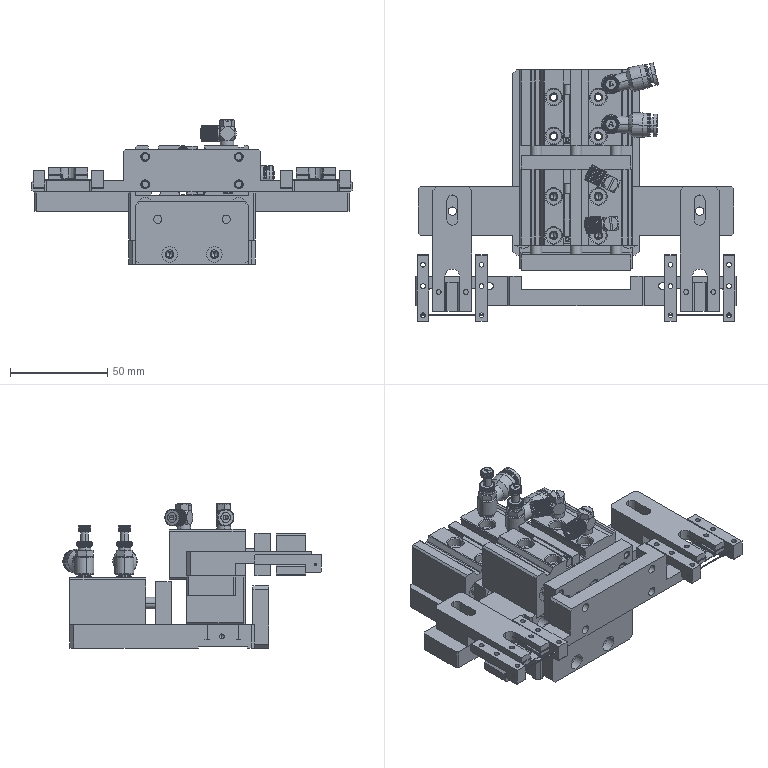Assembly | SolidWorks | mm | 20 component files | 26 solids | 3372 faces | box 165 x 132.62 x 74 mm | volume 291861 mm3 | plane 1468 | cylinder 1040 | cone 830 | torus 20 | sphere 14 | commonest cylinder face diameters 8 x164 6.4 x148 8.5 x72 2.5 x62 3 x50 0.8 x48 6 x40 0.4 x40
Bill of materials:
2018SOLIDWORKS1400000004 | 1 | 45 Steel | Rectangular plate with chamfered corners, a stepped rebate along one long top edge, four large holes near one end, four small holes in a rectangular pattern, and small holes in one side face.
2018SOLIDWORKS1400000005 | 1 | 6061 Alloy | Long rectangular bar with a deeper, wider central block; two end arms each have one through hole, and the central block has four small top holes and four side holes.
2018SOLIDWORKS1400000006 | 2 | 45 Steel | Elongated rectangular block with an open U-shaped fork slot at one end, an oblong slot at the other end, a thin horizontal slit along the forked section, and a deeper stepped portion under the closed end.
2018SOLIDWORKS1400000007 | 1 | Bakelite | Long bar with a raised central rectangular block and thinner arms ending in L-shaped hooked tabs; the central block has four side holes and each arm has a slotted hole and an end hole.
2018SOLIDWORKS1400000008 | 4 | Brass | L-shaped rectangular bar: a long beam with three through holes along its top face and a short downward leg at one end with a small cross hole.
2018SOLIDWORKS1400000024 | 1 | 6061 Alloy | Thick rectangular plate with chamfered corners and four through holes in a trapezoid pattern.
2018SOLIDWORKS1400000501 | 2 | SUS 304 | Composite turned body: a central body with two flat circular faces, a slotted hex on top, a stepped cylindrical spigot below, and a knurled/fluted cylindrical knob extending sideways.
PurchasedPart_MS-5HLH-6StainlessSteelConnector | 2 |  | Formed sheet of uniform thickness with a hat/channel cross-section: two flat flanges and a recessed central channel, with rounded bends and rounded plan corners.
PurchasedPart_ResistanceWireL50 | 2 |  | Slender straight solid cylindrical rod with plain flat ends.
PurchasedPart_Three-axisCylinderTCL12x10S | 2 |  | Rectangular block body joined to a separate end plate by three parallel cylindrical rods; the body has counterbored holes, longitudinal grooves, and side ports/holes.
PurchasedPart_ThrottleValvePSL6M5ABy | 2 |  | Elbow-shaped body made of turned cylinders. A vertical cylindrical body has a hex section near the top. On top of it sit a knurled ring and a smaller knurled cap on a slender stem. A short stepped spigot with a groove sticks out of the bottom. A horizontal cylindrical arm comes off the side of the body and widens through a tapered step into a larger barrel. The barrel ends in a grooved collar and an open circular bore. The overall look matches an elbow flow-control or push-in style pneumatic fitting, but this is not confirmed.
Mates:
1. coincident | 2018SOLIDWORKS1400000007-1 face at (80.712, -88.5, 217) dir (0, 0, 1) | 2018SOLIDWORKS1400000008-2 face at (114.712, -105.5, 217) dir (0, 0, -1)
2. concentric | 2018SOLIDWORKS1400000007-1 face at (84.712, -93.5, 233) dir (0, 0, -1) r 1.6 | 2018SOLIDWORKS1400000008-1 face at (84.712, -93.5, 222) dir (0, 0, 1) r 1.25
3. coincident | 2018SOLIDWORKS1400000007-1 face at (245.712, -88.5, 217) dir (0, 0, 1) | 2018SOLIDWORKS1400000008-3 face at (241.712, -105.5, 217) dir (0, 0, -1)
4. parallel | 2018SOLIDWORKS1400000007-1 face at (80.712, -103.5, 233) dir (-1, 0, 0) | 2018SOLIDWORKS1400000008-1 face at (81.712, -105.5, 215) dir (-1, 0, 0)
5. concentric | 2018SOLIDWORKS1400000007-1 face at (241.712, -93.5, 233) dir (0, 0, -1) r 1.6 | 2018SOLIDWORKS1400000008-3 face at (241.712, -93.5, 222) dir (0, 0, 1) r 1.25
6. concentric | 2018SOLIDWORKS1400000007-1 face at (139.212, -103.5, 229) dir (0, -1, 0) r 2.25 | PurchasedPart_Three-axisCylinderTCL12x10S-1 face at (139.212, -77.5, 229) dir (0, -1, 0) r 1.621
7. concentric | 2018SOLIDWORKS1400000007-1 face at (139.212, -103.5, 215) dir (0, -1, 0) r 2.25 | PurchasedPart_Three-axisCylinderTCL12x10S-1 face at (139.212, -77.5, 215) dir (0, -1, 0) r 1.621
8. distance | 2018SOLIDWORKS1400000007-1 face at (163.212, -95.5, 222) dir (0, 1, 0) | PurchasedPart_Three-axisCylinderTCL12x10S-1 face at (163.212, -85.5, 222) dir (0, -1, 0)
9. concentric | PurchasedPart_ResistanceWireL50-1 face at (81.712, -108.5, 217) dir (1, 0, 0) r 0.3 | 2018SOLIDWORKS1400000008-1 face at (81.712, -108.5, 217) dir (1, 0, 0) r 0.6
10. coincident | PurchasedPart_ResistanceWireL50-1 face at (81.712, -108.5, 217) dir (-1, 0, 0) | 2018SOLIDWORKS1400000008-1 face at (81.712, -105.5, 215) dir (-1, 0, 0)
11. coincident | 2018SOLIDWORKS1400000008-1 face at (87.712, -111.5, 217) dir (0, -1, 0) | 2018SOLIDWORKS1400000008-2 face at (117.712, -111.5, 217) dir (0, -1, 0)
12. concentric | PurchasedPart_ResistanceWireL50-1 face at (81.712, -108.5, 217) dir (1, 0, 0) r 0.3 | 2018SOLIDWORKS1400000008-2 face at (111.712, -108.5, 217) dir (1, 0, 0) r 0.6
13. coincident | 2018SOLIDWORKS1400000008-2 face at (117.712, -105.5, 215) dir (1, 0, 0) | PurchasedPart_ResistanceWireL50-1 face at (117.712, -108.5, 217) dir (1, 0, 0)
14. concentric | 2018SOLIDWORKS1400000008-3 face at (238.712, -108.5, 217) dir (1, 0, 0) r 0.6 | PurchasedPart_ResistanceWireL50-2 face at (208.712, -108.5, 217) dir (1, 0, 0) r 0.3
15. coincident | 2018SOLIDWORKS1400000008-3 face at (244.712, -105.5, 215) dir (1, 0, 0) | PurchasedPart_ResistanceWireL50-2 face at (244.712, -108.5, 217) dir (1, 0, 0)
16. coincident | 2018SOLIDWORKS1400000008-3 face at (244.712, -105.5, 215) dir (1, 0, 0) | PurchasedPart_ResistanceWireL50-2 face at (244.712, -108.5, 217) dir (1, 0, 0)
17. coincident | 2018SOLIDWORKS1400000008-3 face at (244.712, -111.5, 213) dir (0, 0, -1) | 2018SOLIDWORKS1400000008-4 face at (214.712, -111.5, 213) dir (0, 0, -1)
18. concentric | 2018SOLIDWORKS1400000008-4 face at (208.712, -108.5, 217) dir (1, 0, 0) r 0.6 | PurchasedPart_ResistanceWireL50-2 face at (208.712, -108.5, 217) dir (1, 0, 0) r 0.3
19. coincident | 2018SOLIDWORKS1400000008-4 face at (208.712, -105.5, 215) dir (-1, 0, 0) | PurchasedPart_ResistanceWireL50-2 face at (208.712, -108.5, 217) dir (-1, 0, 0)
20. coincident | 2018SOLIDWORKS1400000005-1 face at (163.212, -57.5, 209) dir (0, 0, 1) | PurchasedPart_Three-axisCylinderTCL12x10S-1 face at (156.212, -33.5, 209) dir (0, 0, -1)
21. concentric | 2018SOLIDWORKS1400000005-1 face at (174.712, -67.5, 209) dir (0, 0, 1) r 1.65 | PurchasedPart_Three-axisCylinderTCL12x10S-1 face at (174.712, -67.5, 208.5) dir (0, 0, 1) r 2.25
22. concentric | 2018SOLIDWORKS1400000005-1 face at (151.712, -47.5, 209) dir (0, 0, 1) r 1.65 | PurchasedPart_Three-axisCylinderTCL12x10S-1 face at (151.712, -47.5, 208.5) dir (0, 0, 1) r 2.067
23. coincident | 2018SOLIDWORKS1400000004-1 face at (163.212, -30, 184) dir (0, 0, 1) | PurchasedPart_Three-axisCylinderTCL12x10S-2 face at (156.212, 17.5, 184) dir (0, 0, -1)
24. concentric | 2018SOLIDWORKS1400000004-1 face at (174.712, -16.5, 184) dir (0, 0, 1) r 1.65 | PurchasedPart_Three-axisCylinderTCL12x10S-2 face at (174.712, -16.5, 183.5) dir (0, 0, 1) r 2.25
25. concentric | 2018SOLIDWORKS1400000004-1 face at (151.712, -16.5, 184) dir (0, 0, 1) r 1.65 | PurchasedPart_Three-axisCylinderTCL12x10S-2 face at (151.712, -16.5, 183.5) dir (0, 0, 1) r 2.25
26. distance | 2018SOLIDWORKS1400000005-1 face at (163.212, -44.5, 186) dir (0, 1, 0) | PurchasedPart_Three-axisCylinderTCL12x10S-2 face at (163.212, -34.5, 197) dir (0, -1, 0)
27. concentric | 2018SOLIDWORKS1400000005-1 face at (139.212, -72.5, 204) dir (0, -1, 0) r 2.15 | PurchasedPart_Three-axisCylinderTCL12x10S-2 face at (139.212, -26.5, 204) dir (0, -1, 0) r 1.621
28. concentric | 2018SOLIDWORKS1400000005-1 face at (139.212, -72.5, 190) dir (0, -1, 0) r 2.15 | PurchasedPart_Three-axisCylinderTCL12x10S-2 face at (139.212, -26.5, 190) dir (0, -1, 0) r 1.621
29. width | 2018SOLIDWORKS1400000004-1 face at (192.212, 17.5, 184) dir (-1, 0, 0) | 2018SOLIDWORKS1400000004-1 face at (134.212, 17.5, 184) dir (1, 0, 0) | 2018SOLIDWORKS1400000024-1 face at (134.212, -84.5, 206) dir (-1, 0, 0) | 2018SOLIDWORKS1400000024-1 face at (192.212, -84.5, 206) dir (1, 0, 0)
30. coincident | 2018SOLIDWORKS1400000004-1 face at (163.212, -76.5, 174) dir (0, -1, 0) | 2018SOLIDWORKS1400000024-1 face at (163.212, -76.5, 190) dir (0, 1, 0)
31. coincident | 2018SOLIDWORKS1400000004-1 face at (163.212, -30, 174) dir (0, 0, -1) | 2018SOLIDWORKS1400000024-1 face at (134.212, -84.5, 174) dir (0, 0, -1)
32. width | 2018SOLIDWORKS1400000006-1 face at (89.712, -106.5, 223.5) dir (-1, 0, 0) | 2018SOLIDWORKS1400000006-1 face at (109.712, -106.5, 223.5) dir (1, 0, 0) | 2018SOLIDWORKS1400000501-1 face at (96.212, -99, 218.1) dir (-1, 0, 0) | 2018SOLIDWORKS1400000501-1 face at (103.212, -99, 218.1) dir (1, 0, 0)
33. coincident | 2018SOLIDWORKS1400000006-1 face at (89.712, -106.5, 223.5) dir (0, -1, 0) | 2018SOLIDWORKS1400000501-1 face at (96.212, -106.5, 220.1) dir (0, -1, 0)
34. coincident | 2018SOLIDWORKS1400000006-1 face at (89.712, -86.5, 219.6) dir (0, 0, 1) | 2018SOLIDWORKS1400000501-1 face at (99.712, -99, 219.6) dir (0, 0, -1)
35. coincident | 2018SOLIDWORKS1400000005-1 face at (82.212, -67.5, 211) dir (0, -1, 0) | 2018SOLIDWORKS1400000006-1 face at (89.712, -67.5, 217.6) dir (0, -1, 0)
36. coincident | 2018SOLIDWORKS1400000005-1 face at (163.212, -57.5, 211) dir (0, 0, 1) | 2018SOLIDWORKS1400000006-1 face at (99.712, -74.5, 211) dir (0, 0, -1)
37. width | 2018SOLIDWORKS1400000006-1 face at (102.462, -59.5, 211) dir (-1, 0, 0) | 2018SOLIDWORKS1400000006-1 face at (96.962, -59.5, 211) dir (1, 0, 0) | 2018SOLIDWORKS1400000005-1 face at (99.712, -55, 211) dir (0, 0, 1) r 2.1
38. coincident | 2018SOLIDWORKS1400000006-2 face at (216.712, -106.5, 223.5) dir (0, -1, 0) | 2018SOLIDWORKS1400000501-2 face at (236.212, -106.5, 220.1) dir (0, -1, 0)
39. width | 2018SOLIDWORKS1400000006-2 face at (236.712, -106.5, 223.5) dir (1, 0, 0) | 2018SOLIDWORKS1400000006-2 face at (216.712, -106.5, 223.5) dir (-1, 0, 0) | 2018SOLIDWORKS1400000501-2 face at (230.212, -99, 218.1) dir (1, 0, 0) | 2018SOLIDWORKS1400000501-2 face at (223.212, -99, 218.1) dir (-1, 0, 0)
40. coincident | 2018SOLIDWORKS1400000006-2 face at (216.712, -86.5, 219.6) dir (0, 0, 1) | 2018SOLIDWORKS1400000501-2 face at (226.712, -99, 219.6) dir (0, 0, -1)
41. coincident | 2018SOLIDWORKS1400000005-1 face at (244.212, -67.5, 211) dir (0, -1, 0) | 2018SOLIDWORKS1400000006-2 face at (216.712, -67.5, 217.6) dir (0, -1, 0)
42. coincident | 2018SOLIDWORKS1400000005-1 face at (163.212, -57.5, 211) dir (0, 0, 1) | 2018SOLIDWORKS1400000006-2 face at (226.712, -74.5, 211) dir (0, 0, -1)
43. width | 2018SOLIDWORKS1400000006-2 face at (223.962, -59.5, 211) dir (1, 0, 0) | 2018SOLIDWORKS1400000006-2 face at (229.462, -59.5, 211) dir (-1, 0, 0) | 2018SOLIDWORKS1400000005-1 face at (226.712, -55, 211) dir (0, 0, 1) r 2.1